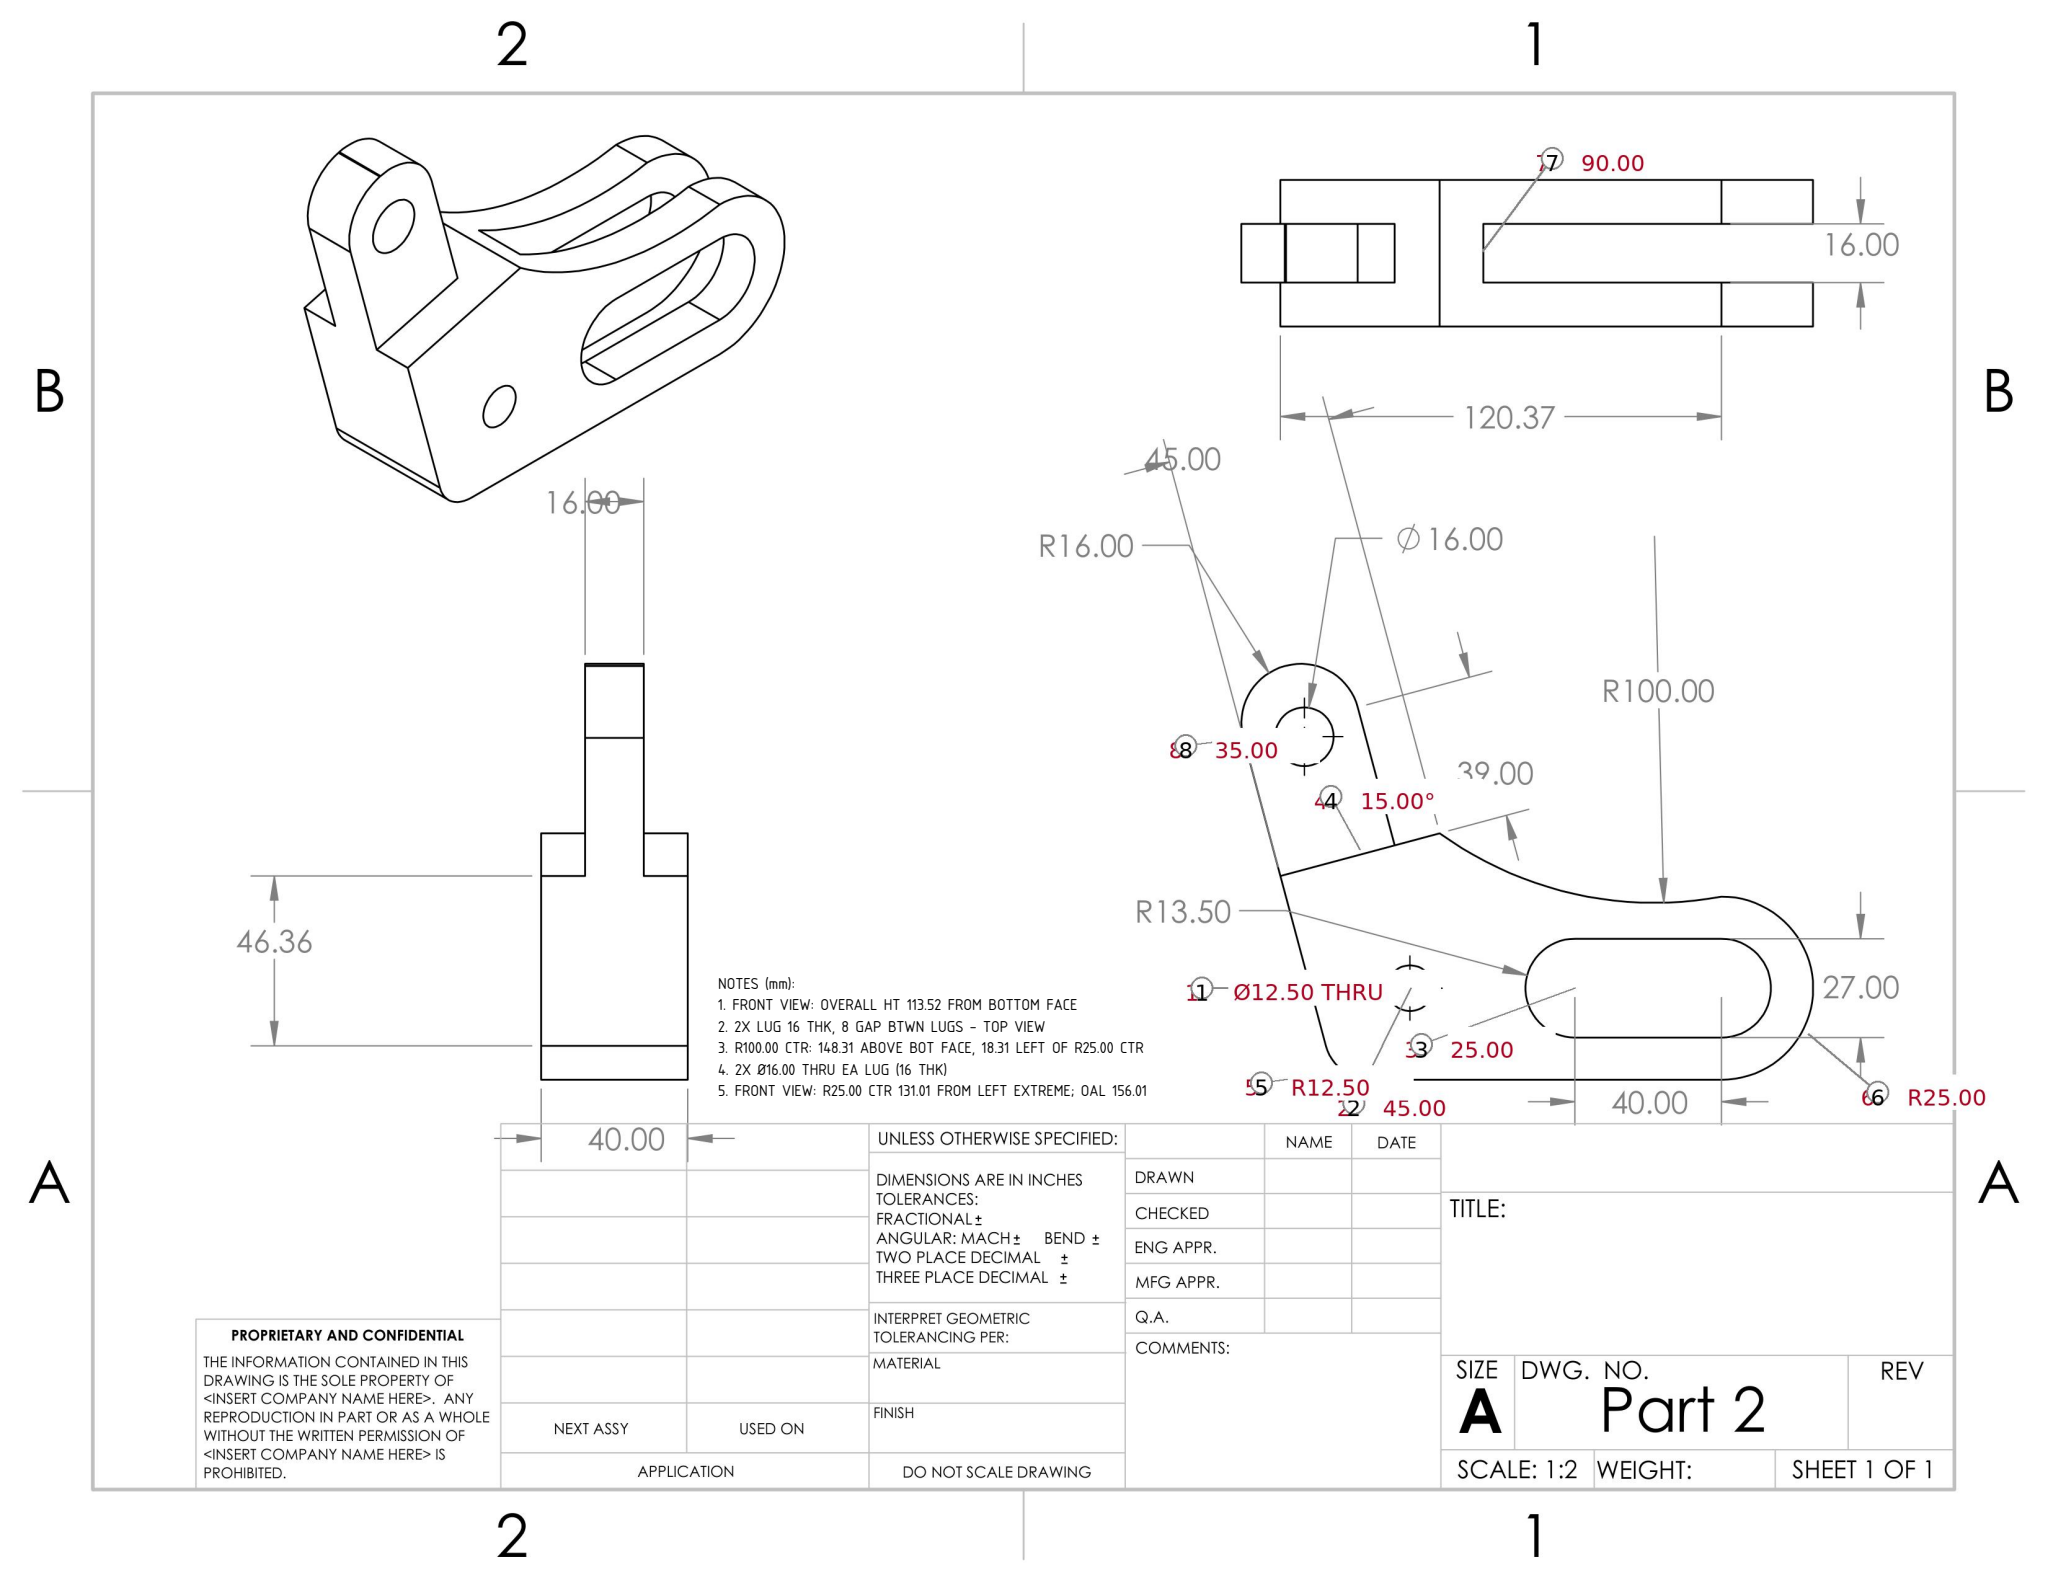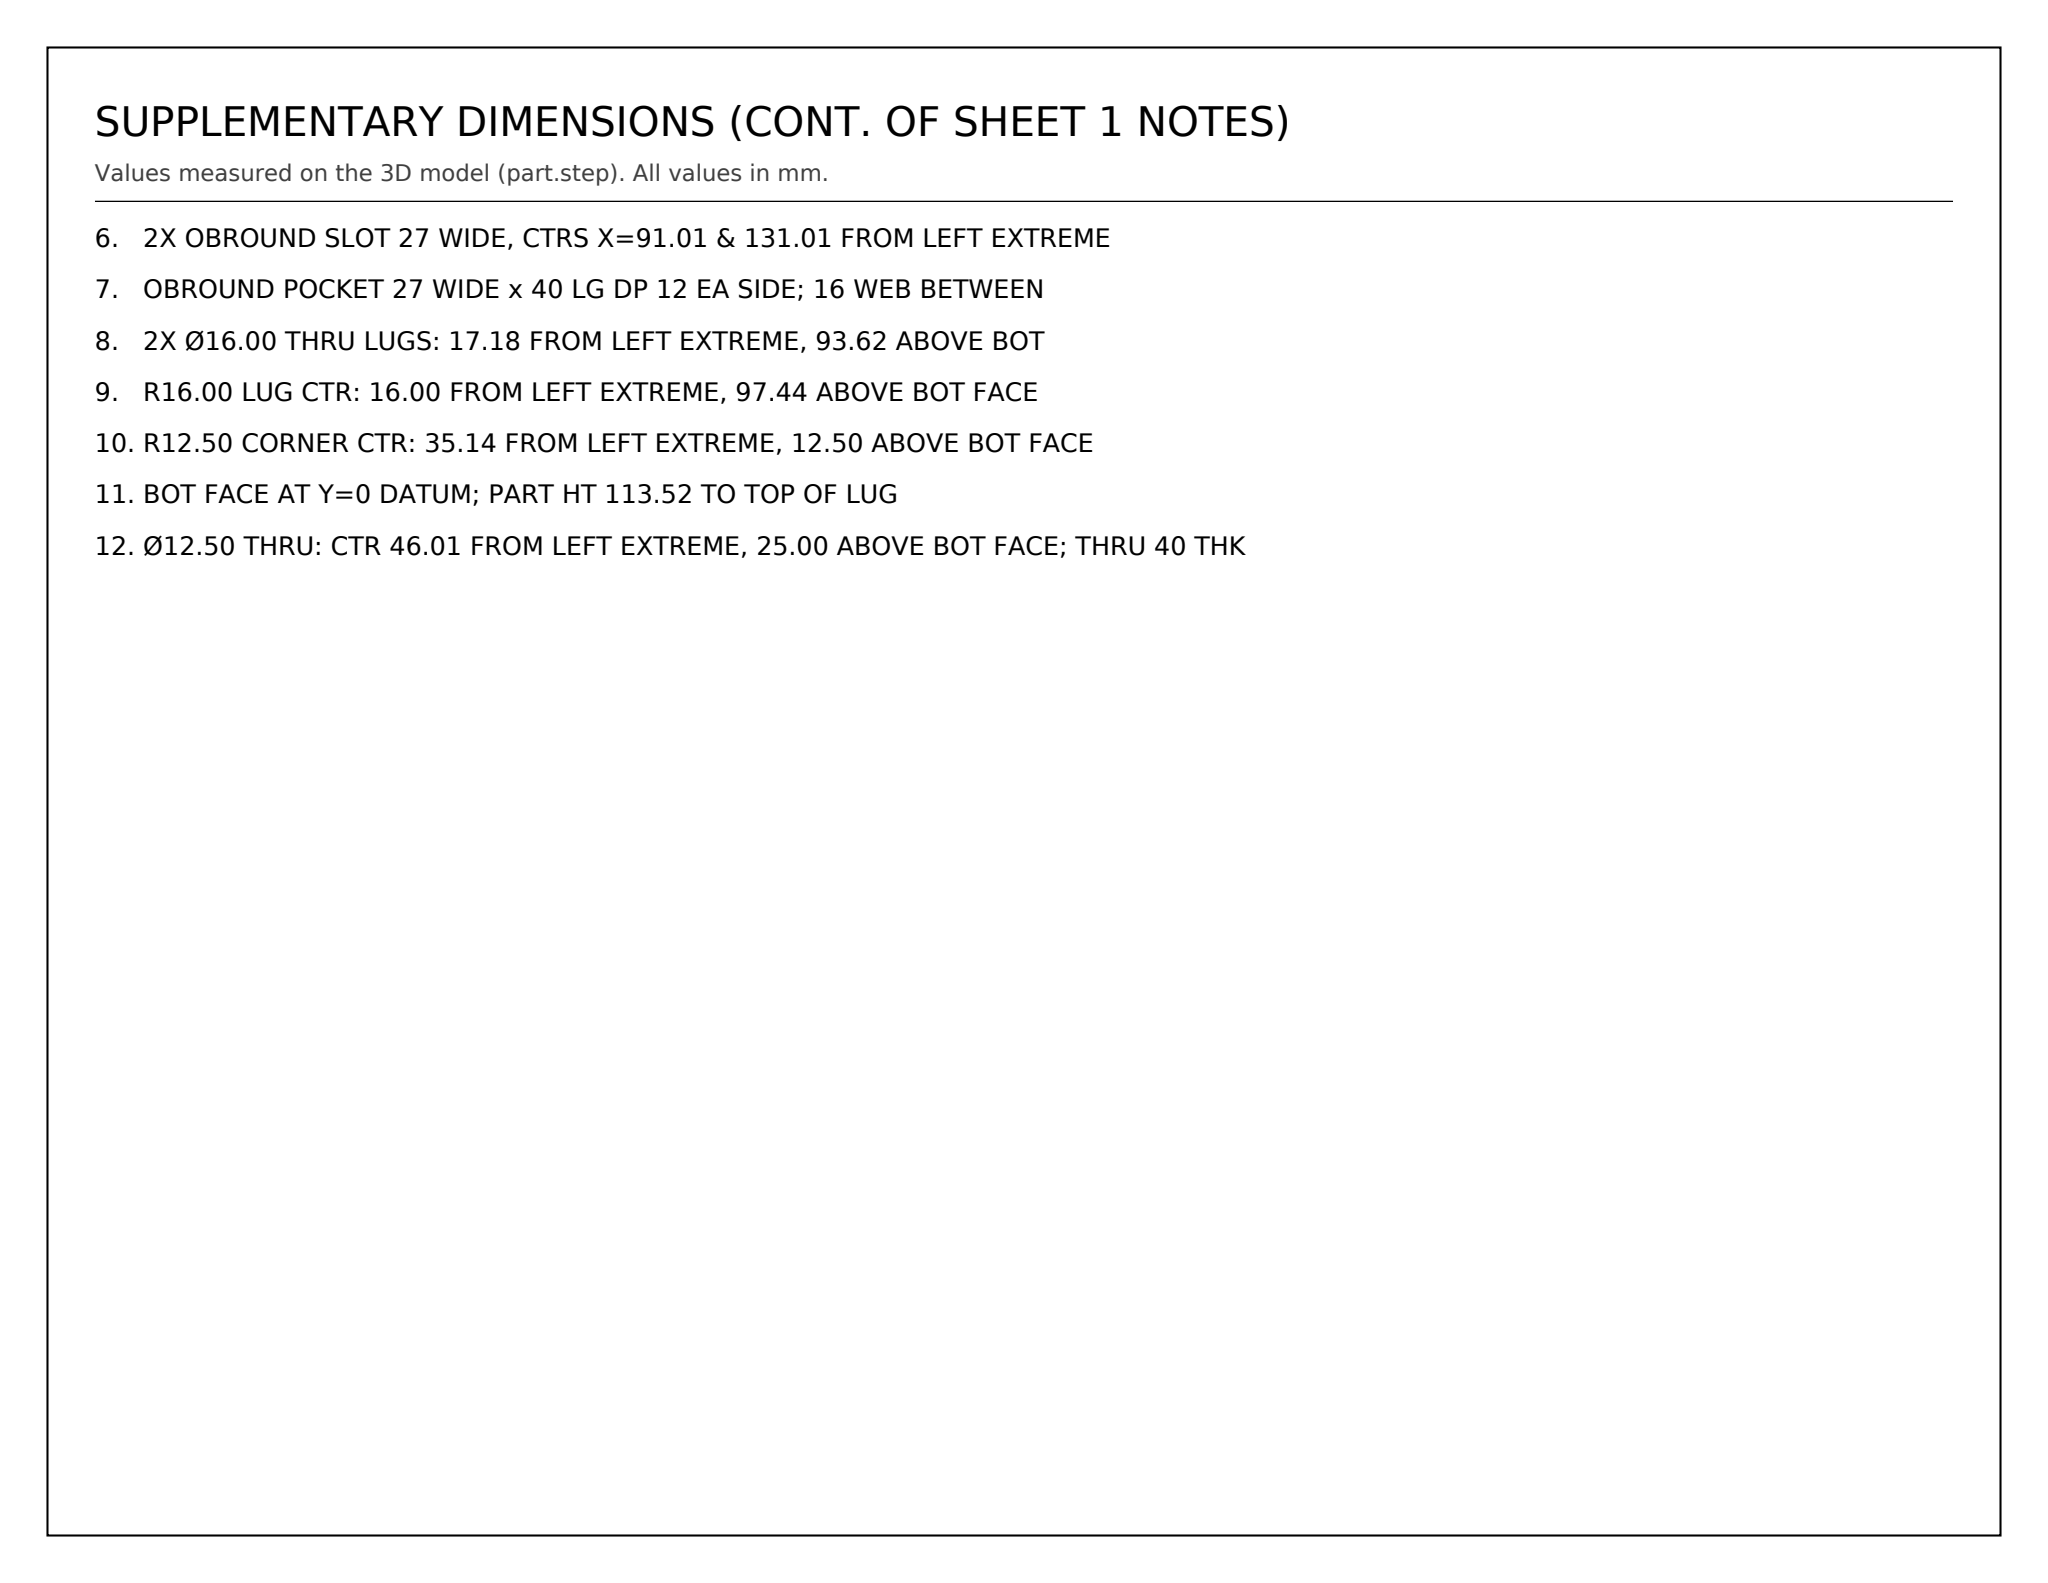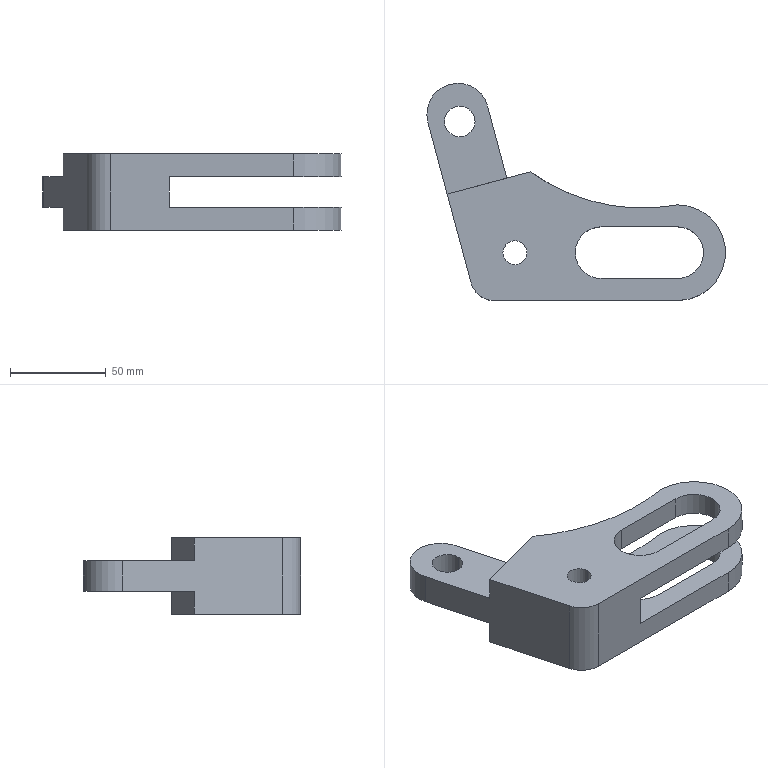Part | SolidWorks | mm | 1 solid | 32 faces | box 156.01 x 113.52 x 40 mm | volume 202005 mm3 | cylinder 16 | plane 16 | commonest cylinder face diameters 27 x6 16 x2 12.5 x2 50 x2 32 x2 25 x1 200 x1
Drawing notes:
FRONT VIEW: OVERALL HT 113.52 FROM BOTTOM FACE | from the solid: bbox_xyz Y = 113.519 (bottom face = y-plane 0.0)
2X LUG 16 THK, 8 GAP BTWN LUGS - TOP VIEW | from the solid: Ø16 and Ø32 lug cyls length 16, qty 2; 16+8+16 = 40 = bbox Z
R100.00 CTR: 148.31 ABOVE BOT FACE, 18.31 LEFT OF R25.00 CTR | from the solid: Ø200 (R100) cyl axis at [112.70,148.31]; R25 end cyl (Ø50) axis at [131.01,25.0]; bottom face y=0
2X Ø16.00 THRU EA LUG (16 THK) | from the solid: cylinders [16.0,'z',[17.18,93.62],len 16, count 2]
FRONT VIEW: R25.00 CTR 131.01 FROM LEFT EXTREME; OAL 156.01 | from the solid: Ø50 cyl axis at x=131.01, y=25.0; bbox_xyz x=156.01 (=131.01+25)
2X OBROUND SLOT 27 WIDE, CTRS X=91.01 & 131.01 FROM LEFT EXTREME | from the solid: Ø27 cyls at (91.01,25) and (131.01,25), 40 apart
OBROUND POCKET 27 WIDE x 40 LG DP 12 EA SIDE; 16 WEB BETWEEN | from the solid: Ø27 cyls length 12; z-planes at 0,12,28,40 (40-28=12, 28-12=16)
2X Ø16.00 THRU LUGS: 17.18 FROM LEFT EXTREME, 93.62 ABOVE BOT | from the solid: Ø16 cyls, axis z, pos (17.18, 93.62), len 16, qty 2
R16.00 LUG CTR: 16.00 FROM LEFT EXTREME, 97.44 ABOVE BOT FACE | from the solid: Ø32 cyl axis at (16.00, 97.44), len 16
R12.50 CORNER CTR: 35.14 FROM LEFT EXTREME, 12.50 ABOVE BOT FACE | from the solid: Ø25 cyl axis at (35.14, 12.5), len 40; y=0 bottom plane
BOT FACE AT Y=0 DATUM; PART HT 113.52 TO TOP OF LUG | from the solid: axis plane y=0.0; bbox_xyz y=113.519
Ø12.50 THRU: CTR 46.01 FROM LEFT EXTREME, 25.00 ABOVE BOT FACE; THRU 40 THK | from the solid: cylinders[dia,axis,pos_other_axes,length]: [12.5,"z",[46.01,25.0,null],40.0] with bbox_xyz [156.01,113.519,40.0], origin at min corner (left extreme / bot face)